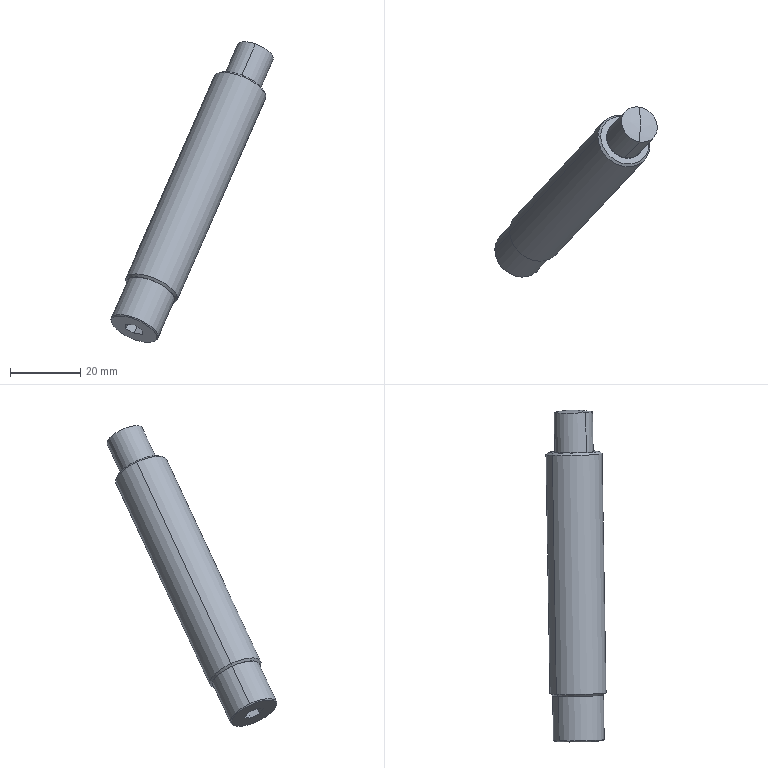Component | SolidWorks | 1369126_DSM_40_270_CC_HD_A_B_0-1_548014_DYSC_12_12_Y1F_SD_0-1 | 1 solid | 32 faces | box 46.37 x 48.48 x 85.78 mm | volume 16355 mm3 | plane 12 | cylinder 10 | cone 8 | sphere 2 | commonest cylinder face diameters 11 x4 6 x2 14.5 x2 16 x2
STEP:
#1=COLOUR_RGB('',0.7922,0.8196,0.9333);
#2=FILL_AREA_STYLE_COLOUR('',#1);
#3=FILL_AREA_STYLE('',(#2));
#4=SURFACE_STYLE_FILL_AREA(#3);
#5=SURFACE_SIDE_STYLE('',(#4));
#6=SURFACE_STYLE_USAGE(.BOTH.,#5);
#7=PRESENTATION_STYLE_ASSIGNMENT((#6));
#8=CARTESIAN_POINT('',(-7.639,80.972,10.386));
#9=VERTEX_POINT('',#8);
#10=CARTESIAN_POINT('',(-7.639,81.364,10.203));
#11=VERTEX_POINT('',#10);
#12=CARTESIAN_POINT('',(-7.639,81.168,10.294));
#13=DIRECTION('',(0.3689,0.3928,0.8424));
#14=DIRECTION('',(0.,-0.9063,0.4226));
#15=AXIS2_PLACEMENT_3D('',#12,#13,#14);
#16=CIRCLE('',#15,0.2165);
#17=EDGE_CURVE('',#9,#11,#16,.T.);
#18=ORIENTED_EDGE('',*,*,#17,.T.);
#19=CARTESIAN_POINT('',(-7.474,81.54,10.58));
#20=VERTEX_POINT('',#19);
#21=CARTESIAN_POINT('',(-7.815,81.177,9.802));
#22=DIRECTION('',(0.3689,0.3928,0.8424));
#23=VECTOR('',#22,39.37);
#24=LINE('',#21,#23);
#25=EDGE_CURVE('',#11,#20,#24,.T.);
#26=ORIENTED_EDGE('',*,*,#25,.T.);
#27=CARTESIAN_POINT('',(-7.474,81.148,10.763));
#28=VERTEX_POINT('',#27);
#29=CARTESIAN_POINT('',(-7.474,81.344,10.671));
#30=DIRECTION('',(0.3689,0.3928,0.8424));
#31=DIRECTION('',(0.,-0.9063,0.4226));
#32=AXIS2_PLACEMENT_3D('',#29,#30,#31);
#33=CIRCLE('',#32,0.2165);
#34=EDGE_CURVE('',#28,#20,#33,.T.);
#35=ORIENTED_EDGE('',*,*,#34,.F.);
#36=CARTESIAN_POINT('',(-7.815,80.785,9.985));
#37=DIRECTION('',(0.3689,0.3928,0.8424));
#38=VECTOR('',#37,39.37);
#39=LINE('',#36,#38);
#40=EDGE_CURVE('',#9,#28,#39,.T.);
#41=ORIENTED_EDGE('',*,*,#40,.F.);
#42=EDGE_LOOP('',(#18,#26,#35,#41));
#43=FACE_OUTER_BOUND('',#42,.T.);
#44=CARTESIAN_POINT('',(-7.815,80.981,9.893));
#45=DIRECTION('',(0.3689,0.3928,0.8424));
#46=DIRECTION('',(0.,-0.9063,0.4226));
#47=AXIS2_PLACEMENT_3D('',#44,#45,#46);
#48=CYLINDRICAL_SURFACE('',#47,0.2165);
#49=ADVANCED_FACE('',(#43),#48,.T.);
#50=CARTESIAN_POINT('',(-7.474,81.344,10.671));
#51=DIRECTION('',(0.3689,0.3928,0.8424));
#52=DIRECTION('',(0.,-0.9063,0.4226));
#53=AXIS2_PLACEMENT_3D('',#50,#51,#52);
#54=CIRCLE('',#53,0.2165);
#55=EDGE_CURVE('',#20,#28,#54,.T.);
#56=ORIENTED_EDGE('',*,*,#55,.T.);
#57=CARTESIAN_POINT('',(-7.465,81.354,10.692));
#58=VERTEX_POINT('',#57);
#59=CARTESIAN_POINT('',(-7.815,80.981,9.893));
#60=DIRECTION('',(-0.9295,0.1559,0.3344));
#61=DIRECTION('',(0.3385,0.,0.941));
#62=AXIS2_PLACEMENT_3D('',#59,#60,#61);
#63=CIRCLE('',#62,0.9488);
#64=EDGE_CURVE('',#28,#58,#63,.T.);
#65=ORIENTED_EDGE('',*,*,#64,.T.);
#66=CARTESIAN_POINT('',(-7.815,80.981,9.893));
#67=DIRECTION('',(0.9295,-0.1559,-0.3344));
#68=DIRECTION('',(-0.3385,0.,-0.941));
#69=AXIS2_PLACEMENT_3D('',#66,#67,#68);
#70=CIRCLE('',#69,0.9488);
#71=EDGE_CURVE('',#20,#58,#70,.T.);
#72=ORIENTED_EDGE('',*,*,#71,.F.);
#73=EDGE_LOOP('',(#56,#65,#72));
#74=FACE_OUTER_BOUND('',#73,.T.);
#75=CARTESIAN_POINT('',(-7.815,80.981,9.893));
#76=DIRECTION('',(-0.9295,0.1559,0.3344));
#77=DIRECTION('',(0.,0.9063,-0.4226));
#78=AXIS2_PLACEMENT_3D('',#75,#76,#77);
#79=SPHERICAL_SURFACE('',#78,0.9488);
#80=ADVANCED_FACE('',(#74),#79,.T.);
#81=CARTESIAN_POINT('',(-7.813,80.875,9.946));
#82=VERTEX_POINT('',#81);
#83=CARTESIAN_POINT('',(-7.813,81.09,9.846));
#84=VERTEX_POINT('',#83);
#85=CARTESIAN_POINT('',(-7.813,80.983,9.896));
#86=DIRECTION('',(0.3689,0.3928,0.8424));
#87=DIRECTION('',(-0.9295,0.1559,0.3344));
#88=AXIS2_PLACEMENT_3D('',#85,#86,#87);
#89=CIRCLE('',#88,0.1181);
#90=EDGE_CURVE('',#82,#84,#89,.T.);
#91=ORIENTED_EDGE('',*,*,#90,.T.);
#92=CARTESIAN_POINT('',(-7.639,81.275,10.244));
#93=VERTEX_POINT('',#92);
#94=CARTESIAN_POINT('',(-7.815,81.088,9.843));
#95=DIRECTION('',(0.3689,0.3928,0.8424));
#96=VECTOR('',#95,39.37);
#97=LINE('',#94,#96);
#98=EDGE_CURVE('',#84,#93,#97,.T.);
#99=ORIENTED_EDGE('',*,*,#98,.T.);
#100=CARTESIAN_POINT('',(-7.639,81.061,10.344));
#101=VERTEX_POINT('',#100);
#102=CARTESIAN_POINT('',(-7.639,81.168,10.294));
#103=DIRECTION('',(0.3689,0.3928,0.8424));
#104=DIRECTION('',(0.,-0.9063,0.4226));
#105=AXIS2_PLACEMENT_3D('',#102,#103,#104);
#106=CIRCLE('',#105,0.1181);
#107=EDGE_CURVE('',#101,#93,#106,.T.);
#108=ORIENTED_EDGE('',*,*,#107,.F.);
#109=CARTESIAN_POINT('',(-7.815,80.874,9.943));
#110=DIRECTION('',(0.3689,0.3928,0.8424));
#111=VECTOR('',#110,39.37);
#112=LINE('',#109,#111);
#113=EDGE_CURVE('',#82,#101,#112,.T.);
#114=ORIENTED_EDGE('',*,*,#113,.F.);
#115=EDGE_LOOP('',(#91,#99,#108,#114));
#116=FACE_OUTER_BOUND('',#115,.T.);
#117=CARTESIAN_POINT('',(-7.815,80.981,9.893));
#118=DIRECTION('',(0.3689,0.3928,0.8424));
#119=DIRECTION('',(0.,-0.9063,0.4226));
#120=AXIS2_PLACEMENT_3D('',#117,#118,#119);
#121=CYLINDRICAL_SURFACE('',#120,0.1181);
#122=ADVANCED_FACE('',(#116),#121,.T.);
#123=CARTESIAN_POINT('',(-8.583,79.85,7.467));
#124=VERTEX_POINT('',#123);
#125=CARTESIAN_POINT('',(-9.092,79.935,7.65));
#126=VERTEX_POINT('',#125);
#127=CARTESIAN_POINT('',(-8.837,79.892,7.558));
#128=DIRECTION('',(0.3689,0.3928,0.8424));
#129=DIRECTION('',(0.9295,-0.1559,-0.3344));
#130=AXIS2_PLACEMENT_3D('',#127,#128,#129);
#131=CIRCLE('',#130,0.2736);
#132=EDGE_CURVE('',#124,#126,#131,.T.);
#133=ORIENTED_EDGE('',*,*,#132,.T.);
#134=CARTESIAN_POINT('',(-9.098,79.941,7.664));
#135=VERTEX_POINT('',#134);
#136=CARTESIAN_POINT('',(-9.092,79.935,7.65));
#137=DIRECTION('',(-0.3963,0.388,0.8321));
#138=VECTOR('',#137,39.37);
#139=LINE('',#136,#138);
#140=EDGE_CURVE('',#126,#135,#139,.T.);
#141=ORIENTED_EDGE('',*,*,#140,.T.);
#142=CARTESIAN_POINT('',(-8.568,79.852,7.473));
#143=VERTEX_POINT('',#142);
#144=CARTESIAN_POINT('',(-8.833,79.897,7.568));
#145=DIRECTION('',(0.3689,0.3928,0.8424));
#146=DIRECTION('',(0.9295,-0.1559,-0.3344));
#147=AXIS2_PLACEMENT_3D('',#144,#145,#146);
#148=CIRCLE('',#147,0.2854);
#149=EDGE_CURVE('',#143,#135,#148,.T.);
#150=ORIENTED_EDGE('',*,*,#149,.F.);
#151=CARTESIAN_POINT('',(-8.583,79.85,7.467));
#152=DIRECTION('',(0.9181,0.1675,0.3592));
#153=VECTOR('',#152,39.37);
#154=LINE('',#151,#153);
#155=EDGE_CURVE('',#124,#143,#154,.T.);
#156=ORIENTED_EDGE('',*,*,#155,.F.);
#157=EDGE_LOOP('',(#133,#141,#150,#156));
#158=FACE_OUTER_BOUND('',#157,.T.);
#159=CARTESIAN_POINT('',(-8.837,79.892,7.558));
#160=DIRECTION('',(0.3689,0.3928,0.8424));
#161=DIRECTION('',(0.9295,-0.1559,-0.3344));
#162=AXIS2_PLACEMENT_3D('',#159,#160,#161);
#163=CONICAL_SURFACE('',#162,0.2736,0.7854);
#164=ADVANCED_FACE('',(#158),#163,.T.);
#165=ORIENTED_EDGE('',*,*,#149,.T.);
#166=CARTESIAN_POINT('',(-8.914,80.138,8.085));
#167=VERTEX_POINT('',#166);
#168=CARTESIAN_POINT('',(-9.103,79.937,7.654));
#169=DIRECTION('',(0.3689,0.3928,0.8424));
#170=VECTOR('',#169,39.37);
#171=LINE('',#168,#170);
#172=EDGE_CURVE('',#135,#167,#171,.T.);
#173=ORIENTED_EDGE('',*,*,#172,.T.);
#174=CARTESIAN_POINT('',(-8.383,80.049,7.894));
#175=VERTEX_POINT('',#174);
#176=CARTESIAN_POINT('',(-8.649,80.093,7.989));
#177=DIRECTION('',(0.3689,0.3928,0.8424));
#178=DIRECTION('',(0.9295,-0.1559,-0.3344));
#179=AXIS2_PLACEMENT_3D('',#176,#177,#178);
#180=CIRCLE('',#179,0.2854);
#181=EDGE_CURVE('',#175,#167,#180,.T.);
#182=ORIENTED_EDGE('',*,*,#181,.F.);
#183=CARTESIAN_POINT('',(-8.572,79.848,7.463));
#184=DIRECTION('',(0.3689,0.3928,0.8424));
#185=VECTOR('',#184,39.37);
#186=LINE('',#183,#185);
#187=EDGE_CURVE('',#143,#175,#186,.T.);
#188=ORIENTED_EDGE('',*,*,#187,.F.);
#189=EDGE_LOOP('',(#165,#173,#182,#188));
#190=FACE_OUTER_BOUND('',#189,.T.);
#191=CARTESIAN_POINT('',(-8.837,79.892,7.558));
#192=DIRECTION('',(0.3689,0.3928,0.8424));
#193=DIRECTION('',(0.9295,-0.1559,-0.3344));
#194=AXIS2_PLACEMENT_3D('',#191,#192,#193);
#195=CYLINDRICAL_SURFACE('',#194,0.2854);
#196=ADVANCED_FACE('',(#190),#195,.T.);
#197=CARTESIAN_POINT('',(-8.378,80.048,7.892));
#198=VERTEX_POINT('',#197);
#199=CARTESIAN_POINT('',(-8.919,80.139,8.087));
#200=VERTEX_POINT('',#199);
#201=CARTESIAN_POINT('',(-8.649,80.093,7.989));
#202=DIRECTION('',(0.3689,0.3928,0.8424));
#203=DIRECTION('',(0.9295,-0.1559,-0.3344));
#204=AXIS2_PLACEMENT_3D('',#201,#202,#203);
#205=CIRCLE('',#204,0.2908);
#206=EDGE_CURVE('',#198,#200,#205,.T.);
#207=ORIENTED_EDGE('',*,*,#206,.T.);
#208=CARTESIAN_POINT('',(-8.932,80.152,8.115));
#209=VERTEX_POINT('',#208);
#210=CARTESIAN_POINT('',(-8.919,80.139,8.087));
#211=DIRECTION('',(-0.3963,0.388,0.8321));
#212=VECTOR('',#211,39.37);
#213=LINE('',#210,#212);
#214=EDGE_CURVE('',#200,#209,#213,.T.);
#215=ORIENTED_EDGE('',*,*,#214,.T.);
#216=CARTESIAN_POINT('',(-8.347,80.054,7.904));
#217=VERTEX_POINT('',#216);
#218=CARTESIAN_POINT('',(-8.64,80.103,8.01));
#219=DIRECTION('',(0.3689,0.3928,0.8424));
#220=DIRECTION('',(0.9295,-0.1559,-0.3344));
#221=AXIS2_PLACEMENT_3D('',#218,#219,#220);
#222=CIRCLE('',#221,0.315);
#223=EDGE_CURVE('',#217,#209,#222,.T.);
#224=ORIENTED_EDGE('',*,*,#223,.F.);
#225=CARTESIAN_POINT('',(-8.378,80.048,7.892));
#226=DIRECTION('',(0.9181,0.1675,0.3592));
#227=VECTOR('',#226,39.37);
#228=LINE('',#225,#227);
#229=EDGE_CURVE('',#198,#217,#228,.T.);
#230=ORIENTED_EDGE('',*,*,#229,.F.);
#231=EDGE_LOOP('',(#207,#215,#224,#230));
#232=FACE_OUTER_BOUND('',#231,.T.);
#233=CARTESIAN_POINT('',(-8.649,80.093,7.989));
#234=DIRECTION('',(0.3689,0.3928,0.8424));
#235=DIRECTION('',(0.9295,-0.1559,-0.3344));
#236=AXIS2_PLACEMENT_3D('',#233,#234,#235);
#237=CONICAL_SURFACE('',#236,0.2908,0.7854);
#238=ADVANCED_FACE('',(#232),#237,.T.);
#239=ORIENTED_EDGE('',*,*,#223,.T.);
#240=CARTESIAN_POINT('',(-7.941,81.208,10.379));
#241=VERTEX_POINT('',#240);
#242=CARTESIAN_POINT('',(-9.13,79.941,7.664));
#243=DIRECTION('',(0.3689,0.3928,0.8424));
#244=VECTOR('',#243,39.37);
#245=LINE('',#242,#244);
#246=EDGE_CURVE('',#209,#241,#245,.T.);
#247=ORIENTED_EDGE('',*,*,#246,.T.);
#248=CARTESIAN_POINT('',(-7.355,81.11,10.169));
#249=VERTEX_POINT('',#248);
#250=CARTESIAN_POINT('',(-7.648,81.159,10.274));
#251=DIRECTION('',(0.3689,0.3928,0.8424));
#252=DIRECTION('',(0.9295,-0.1559,-0.3344));
#253=AXIS2_PLACEMENT_3D('',#250,#251,#252);
#254=CIRCLE('',#253,0.315);
#255=EDGE_CURVE('',#249,#241,#254,.T.);
#256=ORIENTED_EDGE('',*,*,#255,.F.);
#257=CARTESIAN_POINT('',(-8.545,79.843,7.453));
#258=DIRECTION('',(0.3689,0.3928,0.8424));
#259=VECTOR('',#258,39.37);
#260=LINE('',#257,#259);
#261=EDGE_CURVE('',#217,#249,#260,.T.);
#262=ORIENTED_EDGE('',*,*,#261,.F.);
#263=EDGE_LOOP('',(#239,#247,#256,#262));
#264=FACE_OUTER_BOUND('',#263,.T.);
#265=CARTESIAN_POINT('',(-8.837,79.892,7.558));
#266=DIRECTION('',(0.3689,0.3928,0.8424));
#267=DIRECTION('',(0.9295,-0.1559,-0.3344));
#268=AXIS2_PLACEMENT_3D('',#265,#266,#267);
#269=CYLINDRICAL_SURFACE('',#268,0.315);
#270=ADVANCED_FACE('',(#264),#269,.T.);
#271=CARTESIAN_POINT('',(-7.369,81.123,10.197));
#272=VERTEX_POINT('',#271);
#273=CARTESIAN_POINT('',(-7.909,81.213,10.392));
#274=VERTEX_POINT('',#273);
#275=CARTESIAN_POINT('',(-7.639,81.168,10.294));
#276=DIRECTION('',(0.3689,0.3928,0.8424));
#277=DIRECTION('',(0.9295,-0.1559,-0.3344));
#278=AXIS2_PLACEMENT_3D('',#275,#276,#277);
#279=CIRCLE('',#278,0.2908);
#280=EDGE_CURVE('',#272,#274,#279,.T.);
#281=ORIENTED_EDGE('',*,*,#280,.F.);
#282=CARTESIAN_POINT('',(-7.355,81.11,10.169));
#283=DIRECTION('',(0.3963,-0.388,-0.8321));
#284=VECTOR('',#283,39.37);
#285=LINE('',#282,#284);
#286=EDGE_CURVE('',#272,#249,#285,.T.);
#287=ORIENTED_EDGE('',*,*,#286,.T.);
#288=ORIENTED_EDGE('',*,*,#255,.T.);
#289=CARTESIAN_POINT('',(-7.941,81.208,10.379));
#290=DIRECTION('',(-0.9181,-0.1675,-0.3592));
#291=VECTOR('',#290,39.37);
#292=LINE('',#289,#291);
#293=EDGE_CURVE('',#274,#241,#292,.T.);
#294=ORIENTED_EDGE('',*,*,#293,.F.);
#295=EDGE_LOOP('',(#281,#287,#288,#294));
#296=FACE_OUTER_BOUND('',#295,.T.);
#297=CARTESIAN_POINT('',(-7.648,81.159,10.274));
#298=DIRECTION('',(-0.3689,-0.3928,-0.8424));
#299=DIRECTION('',(-0.9295,0.1559,0.3344));
#300=AXIS2_PLACEMENT_3D('',#297,#298,#299);
#301=CONICAL_SURFACE('',#300,0.315,0.7854);
#302=ADVANCED_FACE('',(#296),#301,.T.);
#303=CARTESIAN_POINT('',(-7.842,81.2,10.363));
#304=VERTEX_POINT('',#303);
#305=CARTESIAN_POINT('',(-7.439,81.133,10.219));
#306=VERTEX_POINT('',#305);
#307=CARTESIAN_POINT('',(-7.641,81.167,10.291));
#308=DIRECTION('',(0.3689,0.3928,0.8424));
#309=DIRECTION('',(0.9295,-0.1559,-0.3344));
#310=AXIS2_PLACEMENT_3D('',#307,#308,#309);
#311=CIRCLE('',#310,0.2165);
#312=EDGE_CURVE('',#304,#306,#311,.T.);
#313=ORIENTED_EDGE('',*,*,#312,.F.);
#314=CARTESIAN_POINT('',(-7.844,81.202,10.368));
#315=VERTEX_POINT('',#314);
#316=CARTESIAN_POINT('',(-7.844,81.202,10.368));
#317=DIRECTION('',(-0.3963,0.388,0.8321));
#318=VECTOR('',#317,39.37);
#319=LINE('',#316,#318);
#320=EDGE_CURVE('',#304,#315,#319,.T.);
#321=ORIENTED_EDGE('',*,*,#320,.T.);
#322=CARTESIAN_POINT('',(-7.434,81.134,10.221));
#323=VERTEX_POINT('',#322);
#324=CARTESIAN_POINT('',(-7.639,81.168,10.294));
#325=DIRECTION('',(0.3689,0.3928,0.8424));
#326=DIRECTION('',(0.9295,-0.1559,-0.3344));
#327=AXIS2_PLACEMENT_3D('',#324,#325,#326);
#328=CIRCLE('',#327,0.2205);
#329=EDGE_CURVE('',#315,#323,#328,.T.);
#330=ORIENTED_EDGE('',*,*,#329,.T.);
#331=CARTESIAN_POINT('',(-7.434,81.134,10.221));
#332=DIRECTION('',(0.9181,0.1675,0.3592));
#333=VECTOR('',#332,39.37);
#334=LINE('',#331,#333);
#335=EDGE_CURVE('',#306,#323,#334,.T.);
#336=ORIENTED_EDGE('',*,*,#335,.F.);
#337=EDGE_LOOP('',(#313,#321,#330,#336));
#338=FACE_OUTER_BOUND('',#337,.T.);
#339=CARTESIAN_POINT('',(-7.639,81.168,10.294));
#340=DIRECTION('',(0.3689,0.3928,0.8424));
#341=DIRECTION('',(0.9295,-0.1559,-0.3344));
#342=AXIS2_PLACEMENT_3D('',#339,#340,#341);
#343=CONICAL_SURFACE('',#342,0.2205,0.7854);
#344=ADVANCED_FACE('',(#338),#343,.F.);
#345=CARTESIAN_POINT('',(-8.015,81.016,9.969));
#346=VERTEX_POINT('',#345);
#347=CARTESIAN_POINT('',(-7.612,80.949,9.824));
#348=VERTEX_POINT('',#347);
#349=CARTESIAN_POINT('',(-7.813,80.983,9.896));
#350=DIRECTION('',(0.3689,0.3928,0.8424));
#351=DIRECTION('',(0.9295,-0.1559,-0.3344));
#352=AXIS2_PLACEMENT_3D('',#349,#350,#351);
#353=CIRCLE('',#352,0.2165);
#354=EDGE_CURVE('',#346,#348,#353,.T.);
#355=ORIENTED_EDGE('',*,*,#354,.F.);
#356=CARTESIAN_POINT('',(-9.039,79.926,7.631));
#357=DIRECTION('',(0.3689,0.3928,0.8424));
#358=VECTOR('',#357,39.37);
#359=LINE('',#356,#358);
#360=EDGE_CURVE('',#346,#304,#359,.T.);
#361=ORIENTED_EDGE('',*,*,#360,.T.);
#362=ORIENTED_EDGE('',*,*,#312,.T.);
#363=CARTESIAN_POINT('',(-8.636,79.859,7.486));
#364=DIRECTION('',(0.3689,0.3928,0.8424));
#365=VECTOR('',#364,39.37);
#366=LINE('',#363,#365);
#367=EDGE_CURVE('',#348,#306,#366,.T.);
#368=ORIENTED_EDGE('',*,*,#367,.F.);
#369=EDGE_LOOP('',(#355,#361,#362,#368));
#370=FACE_OUTER_BOUND('',#369,.T.);
#371=CARTESIAN_POINT('',(-8.837,79.892,7.558));
#372=DIRECTION('',(0.3689,0.3928,0.8424));
#373=DIRECTION('',(0.9295,-0.1559,-0.3344));
#374=AXIS2_PLACEMENT_3D('',#371,#372,#373);
#375=CYLINDRICAL_SURFACE('',#374,0.2165);
#376=ADVANCED_FACE('',(#370),#375,.F.);
#377=ORIENTED_EDGE('',*,*,#132,.F.);
#378=CARTESIAN_POINT('',(-8.837,79.892,7.558));
#379=DIRECTION('',(0.3689,0.3928,0.8424));
#380=DIRECTION('',(0.9295,-0.1559,-0.3344));
#381=AXIS2_PLACEMENT_3D('',#378,#379,#380);
#382=CIRCLE('',#381,0.2736);
#383=EDGE_CURVE('',#126,#124,#382,.T.);
#384=ORIENTED_EDGE('',*,*,#383,.F.);
#385=EDGE_LOOP('',(#377,#384));
#386=FACE_OUTER_BOUND('',#385,.T.);
#387=CARTESIAN_POINT('',(-8.837,79.995,7.51));
#388=VERTEX_POINT('',#387);
#389=CARTESIAN_POINT('',(-8.929,79.959,7.567));
#390=VERTEX_POINT('',#389);
#391=CARTESIAN_POINT('',(-8.837,79.995,7.51));
#392=DIRECTION('',(-0.8049,-0.3181,0.5009));
#393=VECTOR('',#392,39.37);
#394=LINE('',#391,#393);
#395=EDGE_CURVE('',#388,#390,#394,.T.);
#396=ORIENTED_EDGE('',*,*,#395,.T.);
#397=CARTESIAN_POINT('',(-8.929,79.856,7.615));
#398=VERTEX_POINT('',#397);
#399=CARTESIAN_POINT('',(-8.929,79.959,7.567));
#400=DIRECTION('',(0.,-0.9063,0.4226));
#401=VECTOR('',#400,39.37);
#402=LINE('',#399,#401);
#403=EDGE_CURVE('',#390,#398,#402,.T.);
#404=ORIENTED_EDGE('',*,*,#403,.T.);
#405=CARTESIAN_POINT('',(-8.837,79.789,7.606));
#406=VERTEX_POINT('',#405);
#407=CARTESIAN_POINT('',(-8.929,79.856,7.615));
#408=DIRECTION('',(0.8049,-0.5882,-0.07826));
#409=VECTOR('',#408,39.37);
#410=LINE('',#407,#409);
#411=EDGE_CURVE('',#398,#406,#410,.T.);
#412=ORIENTED_EDGE('',*,*,#411,.T.);
#413=CARTESIAN_POINT('',(-8.746,79.825,7.549));
#414=VERTEX_POINT('',#413);
#415=CARTESIAN_POINT('',(-8.837,79.789,7.606));
#416=DIRECTION('',(0.8049,0.3181,-0.5009));
#417=VECTOR('',#416,39.37);
#418=LINE('',#415,#417);
#419=EDGE_CURVE('',#406,#414,#418,.T.);
#420=ORIENTED_EDGE('',*,*,#419,.T.);
#421=CARTESIAN_POINT('',(-8.746,79.928,7.501));
#422=VERTEX_POINT('',#421);
#423=CARTESIAN_POINT('',(-8.746,79.825,7.549));
#424=DIRECTION('',(-0.,0.9063,-0.4226));
#425=VECTOR('',#424,39.37);
#426=LINE('',#423,#425);
#427=EDGE_CURVE('',#414,#422,#426,.T.);
#428=ORIENTED_EDGE('',*,*,#427,.T.);
#429=CARTESIAN_POINT('',(-8.746,79.928,7.501));
#430=DIRECTION('',(-0.8049,0.5882,0.07826));
#431=VECTOR('',#430,39.37);
#432=LINE('',#429,#431);
#433=EDGE_CURVE('',#422,#388,#432,.T.);
#434=ORIENTED_EDGE('',*,*,#433,.T.);
#435=EDGE_LOOP('',(#396,#404,#412,#420,#428,#434));
#436=FACE_BOUND('',#435,.T.);
#437=CARTESIAN_POINT('',(-8.837,80.14,7.443));
#438=DIRECTION('',(0.3689,0.3928,0.8424));
#439=DIRECTION('',(0.9295,-0.1559,-0.3344));
#440=AXIS2_PLACEMENT_3D('',#437,#438,#439);
#441=PLANE('',#440);
#442=ADVANCED_FACE('',(#386,#436),#441,.F.);
#443=ORIENTED_EDGE('',*,*,#90,.F.);
#444=CARTESIAN_POINT('',(-7.813,80.983,9.896));
#445=DIRECTION('',(0.3689,0.3928,0.8424));
#446=DIRECTION('',(-0.9295,0.1559,0.3344));
#447=AXIS2_PLACEMENT_3D('',#444,#445,#446);
#448=CIRCLE('',#447,0.1181);
#449=EDGE_CURVE('',#84,#82,#448,.T.);
#450=ORIENTED_EDGE('',*,*,#449,.F.);
#451=EDGE_LOOP('',(#443,#450));
#452=FACE_BOUND('',#451,.T.);
#453=CARTESIAN_POINT('',(-7.813,80.983,9.896));
#454=DIRECTION('',(0.3689,0.3928,0.8424));
#455=DIRECTION('',(0.9295,-0.1559,-0.3344));
#456=AXIS2_PLACEMENT_3D('',#453,#454,#455);
#457=CIRCLE('',#456,0.2165);
#458=EDGE_CURVE('',#348,#346,#457,.T.);
#459=ORIENTED_EDGE('',*,*,#458,.T.);
#460=ORIENTED_EDGE('',*,*,#354,.T.);
#461=EDGE_LOOP('',(#459,#460));
#462=FACE_OUTER_BOUND('',#461,.T.);
#463=CARTESIAN_POINT('',(-7.813,80.983,9.896));
#464=DIRECTION('',(-0.3689,-0.3928,-0.8424));
#465=DIRECTION('',(-0.9295,0.1559,0.3344));
#466=AXIS2_PLACEMENT_3D('',#463,#464,#465);
#467=PLANE('',#466);
#468=ADVANCED_FACE('',(#452,#462),#467,.F.);
#469=ORIENTED_EDGE('',*,*,#360,.F.);
#470=ORIENTED_EDGE('',*,*,#458,.F.);
#471=ORIENTED_EDGE('',*,*,#367,.T.);
#472=CARTESIAN_POINT('',(-7.641,81.167,10.291));
#473=DIRECTION('',(0.3689,0.3928,0.8424));
#474=DIRECTION('',(0.9295,-0.1559,-0.3344));
#475=AXIS2_PLACEMENT_3D('',#472,#473,#474);
#476=CIRCLE('',#475,0.2165);
#477=EDGE_CURVE('',#306,#304,#476,.T.);
#478=ORIENTED_EDGE('',*,*,#477,.T.);
#479=EDGE_LOOP('',(#469,#470,#471,#478));
#480=FACE_OUTER_BOUND('',#479,.T.);
#481=CARTESIAN_POINT('',(-8.837,79.892,7.558));
#482=DIRECTION('',(0.3689,0.3928,0.8424));
#483=DIRECTION('',(0.9295,-0.1559,-0.3344));
#484=AXIS2_PLACEMENT_3D('',#481,#482,#483);
#485=CYLINDRICAL_SURFACE('',#484,0.2165);
#486=ADVANCED_FACE('',(#480),#485,.F.);
#487=ORIENTED_EDGE('',*,*,#320,.F.);
#488=ORIENTED_EDGE('',*,*,#477,.F.);
#489=ORIENTED_EDGE('',*,*,#335,.T.);
#490=CARTESIAN_POINT('',(-7.639,81.168,10.294));
#491=DIRECTION('',(0.3689,0.3928,0.8424));
#492=DIRECTION('',(0.9295,-0.1559,-0.3344));
#493=AXIS2_PLACEMENT_3D('',#490,#491,#492);
#494=CIRCLE('',#493,0.2205);
#495=EDGE_CURVE('',#323,#315,#494,.T.);
#496=ORIENTED_EDGE('',*,*,#495,.T.);
#497=EDGE_LOOP('',(#487,#488,#489,#496));
#498=FACE_OUTER_BOUND('',#497,.T.);
#499=CARTESIAN_POINT('',(-7.639,81.168,10.294));
#500=DIRECTION('',(0.3689,0.3928,0.8424));
#501=DIRECTION('',(0.9295,-0.1559,-0.3344));
#502=AXIS2_PLACEMENT_3D('',#499,#500,#501);
#503=CONICAL_SURFACE('',#502,0.2205,0.7854);
#504=ADVANCED_FACE('',(#498),#503,.F.);
#505=ORIENTED_EDGE('',*,*,#495,.F.);
#506=ORIENTED_EDGE('',*,*,#329,.F.);
#507=EDGE_LOOP('',(#505,#506));
#508=FACE_BOUND('',#507,.T.);
#509=CARTESIAN_POINT('',(-7.639,81.168,10.294));
#510=DIRECTION('',(0.3689,0.3928,0.8424));
#511=DIRECTION('',(0.9295,-0.1559,-0.3344));
#512=AXIS2_PLACEMENT_3D('',#509,#510,#511);
#513=CIRCLE('',#512,0.2908);
#514=EDGE_CURVE('',#274,#272,#513,.T.);
#515=ORIENTED_EDGE('',*,*,#514,.T.);
#516=ORIENTED_EDGE('',*,*,#280,.T.);
#517=EDGE_LOOP('',(#515,#516));
#518=FACE_OUTER_BOUND('',#517,.T.);
#519=CARTESIAN_POINT('',(-7.639,81.368,10.201));
#520=DIRECTION('',(-0.3689,-0.3928,-0.8424));
#521=DIRECTION('',(-0.9295,0.1559,0.3344));
#522=AXIS2_PLACEMENT_3D('',#519,#520,#521);
#523=PLANE('',#522);
#524=ADVANCED_FACE('',(#508,#518),#523,.F.);
#525=ORIENTED_EDGE('',*,*,#286,.F.);
#526=ORIENTED_EDGE('',*,*,#514,.F.);
#527=ORIENTED_EDGE('',*,*,#293,.T.);
#528=CARTESIAN_POINT('',(-7.648,81.159,10.274));
#529=DIRECTION('',(0.3689,0.3928,0.8424));
#530=DIRECTION('',(0.9295,-0.1559,-0.3344));
#531=AXIS2_PLACEMENT_3D('',#528,#529,#530);
#532=CIRCLE('',#531,0.315);
#533=EDGE_CURVE('',#241,#249,#532,.T.);
#534=ORIENTED_EDGE('',*,*,#533,.T.);
#535=EDGE_LOOP('',(#525,#526,#527,#534));
#536=FACE_OUTER_BOUND('',#535,.T.);
#537=CARTESIAN_POINT('',(-7.648,81.159,10.274));
#538=DIRECTION('',(-0.3689,-0.3928,-0.8424));
#539=DIRECTION('',(-0.9295,0.1559,0.3344));
#540=AXIS2_PLACEMENT_3D('',#537,#538,#539);
#541=CONICAL_SURFACE('',#540,0.315,0.7854);
#542=ADVANCED_FACE('',(#536),#541,.T.);
#543=ORIENTED_EDGE('',*,*,#246,.F.);
#544=CARTESIAN_POINT('',(-8.64,80.103,8.01));
#545=DIRECTION('',(0.3689,0.3928,0.8424));
#546=DIRECTION('',(0.9295,-0.1559,-0.3344));
#547=AXIS2_PLACEMENT_3D('',#544,#545,#546);
#548=CIRCLE('',#547,0.315);
#549=EDGE_CURVE('',#209,#217,#548,.T.);
#550=ORIENTED_EDGE('',*,*,#549,.T.);
#551=ORIENTED_EDGE('',*,*,#261,.T.);
#552=ORIENTED_EDGE('',*,*,#533,.F.);
#553=EDGE_LOOP('',(#543,#550,#551,#552));
#554=FACE_OUTER_BOUND('',#553,.T.);
#555=CARTESIAN_POINT('',(-8.837,79.892,7.558));
#556=DIRECTION('',(0.3689,0.3928,0.8424));
#557=DIRECTION('',(0.9295,-0.1559,-0.3344));
#558=AXIS2_PLACEMENT_3D('',#555,#556,#557);
#559=CYLINDRICAL_SURFACE('',#558,0.315);
#560=ADVANCED_FACE('',(#554),#559,.T.);
#561=ORIENTED_EDGE('',*,*,#214,.F.);
#562=CARTESIAN_POINT('',(-8.649,80.093,7.989));
#563=DIRECTION('',(0.3689,0.3928,0.8424));
#564=DIRECTION('',(0.9295,-0.1559,-0.3344));
#565=AXIS2_PLACEMENT_3D('',#562,#563,#564);
#566=CIRCLE('',#565,0.2908);
#567=EDGE_CURVE('',#200,#198,#566,.T.);
#568=ORIENTED_EDGE('',*,*,#567,.T.);
#569=ORIENTED_EDGE('',*,*,#229,.T.);
#570=ORIENTED_EDGE('',*,*,#549,.F.);
#571=EDGE_LOOP('',(#561,#568,#569,#570));
#572=FACE_OUTER_BOUND('',#571,.T.);
#573=CARTESIAN_POINT('',(-8.649,80.093,7.989));
#574=DIRECTION('',(0.3689,0.3928,0.8424));
#575=DIRECTION('',(0.9295,-0.1559,-0.3344));
#576=AXIS2_PLACEMENT_3D('',#573,#574,#575);
#577=CONICAL_SURFACE('',#576,0.2908,0.7854);
#578=ADVANCED_FACE('',(#572),#577,.T.);
#579=ORIENTED_EDGE('',*,*,#206,.F.);
#580=ORIENTED_EDGE('',*,*,#567,.F.);
#581=EDGE_LOOP('',(#579,#580));
#582=FACE_OUTER_BOUND('',#581,.T.);
#583=ORIENTED_EDGE('',*,*,#181,.T.);
#584=CARTESIAN_POINT('',(-8.649,80.093,7.989));
#585=DIRECTION('',(0.3689,0.3928,0.8424));
#586=DIRECTION('',(0.9295,-0.1559,-0.3344));
#587=AXIS2_PLACEMENT_3D('',#584,#585,#586);
#588=CIRCLE('',#587,0.2854);
#589=EDGE_CURVE('',#167,#175,#588,.T.);
#590=ORIENTED_EDGE('',*,*,#589,.T.);
#591=EDGE_LOOP('',(#583,#590));
#592=FACE_BOUND('',#591,.T.);
#593=CARTESIAN_POINT('',(-8.649,80.357,7.866));
#594=DIRECTION('',(0.3689,0.3928,0.8424));
#595=DIRECTION('',(0.9295,-0.1559,-0.3344));
#596=AXIS2_PLACEMENT_3D('',#593,#594,#595);
#597=PLANE('',#596);
#598=ADVANCED_FACE('',(#582,#592),#597,.F.);
#599=ORIENTED_EDGE('',*,*,#172,.F.);
#600=CARTESIAN_POINT('',(-8.833,79.897,7.568));
#601=DIRECTION('',(0.3689,0.3928,0.8424));
#602=DIRECTION('',(0.9295,-0.1559,-0.3344));
#603=AXIS2_PLACEMENT_3D('',#600,#601,#602);
#604=CIRCLE('',#603,0.2854);
#605=EDGE_CURVE('',#135,#143,#604,.T.);
#606=ORIENTED_EDGE('',*,*,#605,.T.);
#607=ORIENTED_EDGE('',*,*,#187,.T.);
#608=ORIENTED_EDGE('',*,*,#589,.F.);
#609=EDGE_LOOP('',(#599,#606,#607,#608));
#610=FACE_OUTER_BOUND('',#609,.T.);
#611=CARTESIAN_POINT('',(-8.837,79.892,7.558));
#612=DIRECTION('',(0.3689,0.3928,0.8424));
#613=DIRECTION('',(0.9295,-0.1559,-0.3344));
#614=AXIS2_PLACEMENT_3D('',#611,#612,#613);
#615=CYLINDRICAL_SURFACE('',#614,0.2854);
#616=ADVANCED_FACE('',(#610),#615,.T.);
#617=ORIENTED_EDGE('',*,*,#140,.F.);
#618=ORIENTED_EDGE('',*,*,#383,.T.);
#619=ORIENTED_EDGE('',*,*,#155,.T.);
#620=ORIENTED_EDGE('',*,*,#605,.F.);
#621=EDGE_LOOP('',(#617,#618,#619,#620));
#622=FACE_OUTER_BOUND('',#621,.T.);
#623=CARTESIAN_POINT('',(-8.837,79.892,7.558));
#624=DIRECTION('',(0.3689,0.3928,0.8424));
#625=DIRECTION('',(0.9295,-0.1559,-0.3344));
#626=AXIS2_PLACEMENT_3D('',#623,#624,#625);
#627=CONICAL_SURFACE('',#626,0.2736,0.7854);
#628=ADVANCED_FACE('',(#622),#627,.T.);
#629=ORIENTED_EDGE('',*,*,#98,.F.);
#630=ORIENTED_EDGE('',*,*,#449,.T.);
#631=ORIENTED_EDGE('',*,*,#113,.T.);
#632=CARTESIAN_POINT('',(-7.639,81.168,10.294));
#633=DIRECTION('',(0.3689,0.3928,0.8424));
#634=DIRECTION('',(0.,-0.9063,0.4226));
#635=AXIS2_PLACEMENT_3D('',#632,#633,#634);
#636=CIRCLE('',#635,0.1181);
#637=EDGE_CURVE('',#93,#101,#636,.T.);
#638=ORIENTED_EDGE('',*,*,#637,.F.);
#639=EDGE_LOOP('',(#629,#630,#631,#638));
#640=FACE_OUTER_BOUND('',#639,.T.);
#641=CARTESIAN_POINT('',(-7.815,80.981,9.893));
#642=DIRECTION('',(0.3689,0.3928,0.8424));
#643=DIRECTION('',(0.,-0.9063,0.4226));
#644=AXIS2_PLACEMENT_3D('',#641,#642,#643);
#645=CYLINDRICAL_SURFACE('',#644,0.1181);
#646=ADVANCED_FACE('',(#640),#645,.T.);
#647=ORIENTED_EDGE('',*,*,#64,.F.);
#648=ORIENTED_EDGE('',*,*,#34,.T.);
#649=ORIENTED_EDGE('',*,*,#71,.T.);
#650=EDGE_LOOP('',(#647,#648,#649));
#651=FACE_OUTER_BOUND('',#650,.T.);
#652=CARTESIAN_POINT('',(-7.815,80.981,9.893));
#653=DIRECTION('',(-0.9295,0.1559,0.3344));
#654=DIRECTION('',(0.,0.9063,-0.4226));
#655=AXIS2_PLACEMENT_3D('',#652,#653,#654);
#656=SPHERICAL_SURFACE('',#655,0.9488);
#657=ADVANCED_FACE('',(#651),#656,.T.);
#658=ORIENTED_EDGE('',*,*,#25,.F.);
#659=CARTESIAN_POINT('',(-7.639,81.168,10.294));
#660=DIRECTION('',(0.3689,0.3928,0.8424));
#661=DIRECTION('',(0.,-0.9063,0.4226));
#662=AXIS2_PLACEMENT_3D('',#659,#660,#661);
#663=CIRCLE('',#662,0.2165);
#664=EDGE_CURVE('',#11,#9,#663,.T.);
#665=ORIENTED_EDGE('',*,*,#664,.T.);
#666=ORIENTED_EDGE('',*,*,#40,.T.);
#667=ORIENTED_EDGE('',*,*,#55,.F.);
#668=EDGE_LOOP('',(#658,#665,#666,#667));
#669=FACE_OUTER_BOUND('',#668,.T.);
#670=CARTESIAN_POINT('',(-7.815,80.981,9.893));
#671=DIRECTION('',(0.3689,0.3928,0.8424));
#672=DIRECTION('',(0.,-0.9063,0.4226));
#673=AXIS2_PLACEMENT_3D('',#670,#671,#672);
#674=CYLINDRICAL_SURFACE('',#673,0.2165);
#675=ADVANCED_FACE('',(#669),#674,.T.);
#676=ORIENTED_EDGE('',*,*,#17,.F.);
#677=ORIENTED_EDGE('',*,*,#664,.F.);
#678=EDGE_LOOP('',(#676,#677));
#679=FACE_OUTER_BOUND('',#678,.T.);
#680=ORIENTED_EDGE('',*,*,#107,.T.);
#681=ORIENTED_EDGE('',*,*,#637,.T.);
#682=EDGE_LOOP('',(#680,#681));
#683=FACE_BOUND('',#682,.T.);
#684=CARTESIAN_POINT('',(-7.639,81.364,10.203));
#685=DIRECTION('',(0.3689,0.3928,0.8424));
#686=DIRECTION('',(-0.,-0.9063,0.4226));
#687=AXIS2_PLACEMENT_3D('',#684,#685,#686);
#688=PLANE('',#687);
#689=ADVANCED_FACE('',(#679,#683),#688,.F.);
#690=ORIENTED_EDGE('',*,*,#395,.F.);
#691=CARTESIAN_POINT('',(-8.801,80.034,7.593));
#692=VERTEX_POINT('',#691);
#693=CARTESIAN_POINT('',(-8.801,80.034,7.593));
#694=DIRECTION('',(-0.3689,-0.3928,-0.8424));
#695=VECTOR('',#694,39.37);
#696=LINE('',#693,#695);
#697=EDGE_CURVE('',#692,#388,#696,.T.);
#698=ORIENTED_EDGE('',*,*,#697,.F.);
#699=CARTESIAN_POINT('',(-8.893,79.998,7.65));
#700=VERTEX_POINT('',#699);
#701=CARTESIAN_POINT('',(-8.801,80.034,7.593));
#702=DIRECTION('',(-0.8049,-0.3181,0.5009));
#703=VECTOR('',#702,39.37);
#704=LINE('',#701,#703);
#705=EDGE_CURVE('',#692,#700,#704,.T.);
#706=ORIENTED_EDGE('',*,*,#705,.T.);
#707=CARTESIAN_POINT('',(-8.893,79.998,7.65));
#708=DIRECTION('',(-0.3689,-0.3928,-0.8424));
#709=VECTOR('',#708,39.37);
#710=LINE('',#707,#709);
#711=EDGE_CURVE('',#700,#390,#710,.T.);
#712=ORIENTED_EDGE('',*,*,#711,.T.);
#713=EDGE_LOOP('',(#690,#698,#706,#712));
#714=FACE_OUTER_BOUND('',#713,.T.);
#715=CARTESIAN_POINT('',(-8.801,80.034,7.593));
#716=DIRECTION('',(0.4647,-0.8628,0.1988));
#717=DIRECTION('',(0.8049,0.3181,-0.5009));
#718=AXIS2_PLACEMENT_3D('',#715,#716,#717);
#719=PLANE('',#718);
#720=ADVANCED_FACE('',(#714),#719,.T.);
#721=ORIENTED_EDGE('',*,*,#403,.F.);
#722=ORIENTED_EDGE('',*,*,#711,.F.);
#723=CARTESIAN_POINT('',(-8.893,79.895,7.698));
#724=VERTEX_POINT('',#723);
#725=CARTESIAN_POINT('',(-8.893,79.998,7.65));
#726=DIRECTION('',(0.,-0.9063,0.4226));
#727=VECTOR('',#726,39.37);
#728=LINE('',#725,#727);
#729=EDGE_CURVE('',#700,#724,#728,.T.);
#730=ORIENTED_EDGE('',*,*,#729,.T.);
#731=CARTESIAN_POINT('',(-8.893,79.895,7.698));
#732=DIRECTION('',(-0.3689,-0.3928,-0.8424));
#733=VECTOR('',#732,39.37);
#734=LINE('',#731,#733);
#735=EDGE_CURVE('',#724,#398,#734,.T.);
#736=ORIENTED_EDGE('',*,*,#735,.T.);
#737=EDGE_LOOP('',(#721,#722,#730,#736));
#738=FACE_OUTER_BOUND('',#737,.T.);
#739=CARTESIAN_POINT('',(-8.893,79.998,7.65));
#740=DIRECTION('',(0.9295,-0.1559,-0.3344));
#741=DIRECTION('',(-0.3689,-0.3928,-0.8424));
#742=AXIS2_PLACEMENT_3D('',#739,#740,#741);
#743=PLANE('',#742);
#744=ADVANCED_FACE('',(#738),#743,.T.);
#745=ORIENTED_EDGE('',*,*,#411,.F.);
#746=ORIENTED_EDGE('',*,*,#735,.F.);
#747=CARTESIAN_POINT('',(-8.801,79.828,7.689));
#748=VERTEX_POINT('',#747);
#749=CARTESIAN_POINT('',(-8.893,79.895,7.698));
#750=DIRECTION('',(0.8049,-0.5882,-0.07826));
#751=VECTOR('',#750,39.37);
#752=LINE('',#749,#751);
#753=EDGE_CURVE('',#724,#748,#752,.T.);
#754=ORIENTED_EDGE('',*,*,#753,.T.);
#755=CARTESIAN_POINT('',(-8.801,79.828,7.689));
#756=DIRECTION('',(-0.3689,-0.3928,-0.8424));
#757=VECTOR('',#756,39.37);
#758=LINE('',#755,#757);
#759=EDGE_CURVE('',#748,#406,#758,.T.);
#760=ORIENTED_EDGE('',*,*,#759,.T.);
#761=EDGE_LOOP('',(#745,#746,#754,#760));
#762=FACE_OUTER_BOUND('',#761,.T.);
#763=CARTESIAN_POINT('',(-8.893,79.895,7.698));
#764=DIRECTION('',(0.4647,0.7069,-0.5332));
#765=DIRECTION('',(-0.8049,0.5882,0.07826));
#766=AXIS2_PLACEMENT_3D('',#763,#764,#765);
#767=PLANE('',#766);
#768=ADVANCED_FACE('',(#762),#767,.T.);
#769=ORIENTED_EDGE('',*,*,#419,.F.);
#770=ORIENTED_EDGE('',*,*,#759,.F.);
#771=CARTESIAN_POINT('',(-8.71,79.864,7.632));
#772=VERTEX_POINT('',#771);
#773=CARTESIAN_POINT('',(-8.801,79.828,7.689));
#774=DIRECTION('',(0.8049,0.3181,-0.5009));
#775=VECTOR('',#774,39.37);
#776=LINE('',#773,#775);
#777=EDGE_CURVE('',#748,#772,#776,.T.);
#778=ORIENTED_EDGE('',*,*,#777,.T.);
#779=CARTESIAN_POINT('',(-8.71,79.864,7.632));
#780=DIRECTION('',(-0.3689,-0.3928,-0.8424));
#781=VECTOR('',#780,39.37);
#782=LINE('',#779,#781);
#783=EDGE_CURVE('',#772,#414,#782,.T.);
#784=ORIENTED_EDGE('',*,*,#783,.T.);
#785=EDGE_LOOP('',(#769,#770,#778,#784));
#786=FACE_OUTER_BOUND('',#785,.T.);
#787=CARTESIAN_POINT('',(-8.801,79.828,7.689));
#788=DIRECTION('',(-0.4647,0.8628,-0.1988));
#789=DIRECTION('',(-0.8049,-0.3181,0.5009));
#790=AXIS2_PLACEMENT_3D('',#787,#788,#789);
#791=PLANE('',#790);
#792=ADVANCED_FACE('',(#786),#791,.T.);
#793=ORIENTED_EDGE('',*,*,#427,.F.);
#794=ORIENTED_EDGE('',*,*,#783,.F.);
#795=CARTESIAN_POINT('',(-8.71,79.967,7.584));
#796=VERTEX_POINT('',#795);
#797=CARTESIAN_POINT('',(-8.71,79.864,7.632));
#798=DIRECTION('',(-0.,0.9063,-0.4226));
#799=VECTOR('',#798,39.37);
#800=LINE('',#797,#799);
#801=EDGE_CURVE('',#772,#796,#800,.T.);
#802=ORIENTED_EDGE('',*,*,#801,.T.);
#803=CARTESIAN_POINT('',(-8.71,79.967,7.584));
#804=DIRECTION('',(-0.3689,-0.3928,-0.8424));
#805=VECTOR('',#804,39.37);
#806=LINE('',#803,#805);
#807=EDGE_CURVE('',#796,#422,#806,.T.);
#808=ORIENTED_EDGE('',*,*,#807,.T.);
#809=EDGE_LOOP('',(#793,#794,#802,#808));
#810=FACE_OUTER_BOUND('',#809,.T.);
#811=CARTESIAN_POINT('',(-8.71,79.864,7.632));
#812=DIRECTION('',(-0.9295,0.1559,0.3344));
#813=DIRECTION('',(0.3689,0.3928,0.8424));
#814=AXIS2_PLACEMENT_3D('',#811,#812,#813);
#815=PLANE('',#814);
#816=ADVANCED_FACE('',(#810),#815,.T.);
#817=ORIENTED_EDGE('',*,*,#433,.F.);
#818=ORIENTED_EDGE('',*,*,#807,.F.);
#819=CARTESIAN_POINT('',(-8.71,79.967,7.584));
#820=DIRECTION('',(-0.8049,0.5882,0.07826));
#821=VECTOR('',#820,39.37);
#822=LINE('',#819,#821);
#823=EDGE_CURVE('',#796,#692,#822,.T.);
#824=ORIENTED_EDGE('',*,*,#823,.T.);
#825=ORIENTED_EDGE('',*,*,#697,.T.);
#826=EDGE_LOOP('',(#817,#818,#824,#825));
#827=FACE_OUTER_BOUND('',#826,.T.);
#828=CARTESIAN_POINT('',(-8.71,79.967,7.584));
#829=DIRECTION('',(-0.4647,-0.7069,0.5332));
#830=DIRECTION('',(0.8049,-0.5882,-0.07826));
#831=AXIS2_PLACEMENT_3D('',#828,#829,#830);
#832=PLANE('',#831);
#833=ADVANCED_FACE('',(#827),#832,.T.);
#834=ORIENTED_EDGE('',*,*,#705,.F.);
#835=ORIENTED_EDGE('',*,*,#823,.F.);
#836=ORIENTED_EDGE('',*,*,#801,.F.);
#837=ORIENTED_EDGE('',*,*,#777,.F.);
#838=ORIENTED_EDGE('',*,*,#753,.F.);
#839=ORIENTED_EDGE('',*,*,#729,.F.);
#840=EDGE_LOOP('',(#834,#835,#836,#837,#838,#839));
#841=FACE_OUTER_BOUND('',#840,.T.);
#842=CARTESIAN_POINT('',(-8.801,79.931,7.641));
#843=DIRECTION('',(0.3689,0.3928,0.8424));
#844=DIRECTION('',(0.9295,-0.1559,-0.3344));
#845=AXIS2_PLACEMENT_3D('',#842,#843,#844);
#846=PLANE('',#845);
#847=ADVANCED_FACE('',(#841),#846,.F.);
#848=CLOSED_SHELL('',(#49,#80,#122,#164,#196,#238,#270,#302,#344,#376,#442,#468,#486,#504,#524,#542,#560,#578,#598,#616,#628,#646,#657,#675,#689,#720,#744,#768,#792,#816,#833,#847));
#849=MANIFOLD_SOLID_BREP('',#848);
#850=STYLED_ITEM('',(#7),#849);
#851=(LENGTH_UNIT()NAMED_UNIT(*)SI_UNIT($,.METRE.));
#852=LENGTH_MEASURE_WITH_UNIT(LENGTH_MEASURE(0.0254),#851);
#853=DIMENSIONAL_EXPONENTS(1.,0.,0.,0.,0.,0.,0.);
#854=(CONVERSION_BASED_UNIT('',#852)LENGTH_UNIT()NAMED_UNIT(#853));
#855=UNCERTAINTY_MEASURE_WITH_UNIT(LENGTH_MEASURE(0.00001),#854,'','');
#856=(NAMED_UNIT(*)PLANE_ANGLE_UNIT()SI_UNIT($,.RADIAN.));
#857=(NAMED_UNIT(*)SI_UNIT($,.STERADIAN.)SOLID_ANGLE_UNIT());
#858=(GEOMETRIC_REPRESENTATION_CONTEXT(3)GLOBAL_UNCERTAINTY_ASSIGNED_CONTEXT((#855))GLOBAL_UNIT_ASSIGNED_CONTEXT((#854,#856,#857))REPRESENTATION_CONTEXT('',''));
#859=MECHANICAL_DESIGN_GEOMETRIC_PRESENTATION_REPRESENTATION('',(#850),#858);
#860=CARTESIAN_POINT('',(0.,0.,0.));
#861=DIRECTION('',(0.,0.,1.));
#862=DIRECTION('',(1.,0.,0.));
#863=AXIS2_PLACEMENT_3D('',#860,#861,#862);
#864=(LENGTH_UNIT()NAMED_UNIT(*)SI_UNIT($,.METRE.));
#865=LENGTH_MEASURE_WITH_UNIT(LENGTH_MEASURE(0.0254),#864);
#866=DIMENSIONAL_EXPONENTS(1.,0.,0.,0.,0.,0.,0.);
#867=(CONVERSION_BASED_UNIT('',#865)LENGTH_UNIT()NAMED_UNIT(#866));
#868=UNCERTAINTY_MEASURE_WITH_UNIT(LENGTH_MEASURE(0.00001),#867,'','');
#869=(NAMED_UNIT(*)PLANE_ANGLE_UNIT()SI_UNIT($,.RADIAN.));
#870=(NAMED_UNIT(*)SI_UNIT($,.STERADIAN.)SOLID_ANGLE_UNIT());
#871=(GEOMETRIC_REPRESENTATION_CONTEXT(3)GLOBAL_UNCERTAINTY_ASSIGNED_CONTEXT((#868))GLOBAL_UNIT_ASSIGNED_CONTEXT((#867,#869,#870))REPRESENTATION_CONTEXT('',''));
#872=ADVANCED_BREP_SHAPE_REPRESENTATION('',(#849,#863),#871);
#873=PRESENTATION_LAYER_ASSIGNMENT('','',(#850));